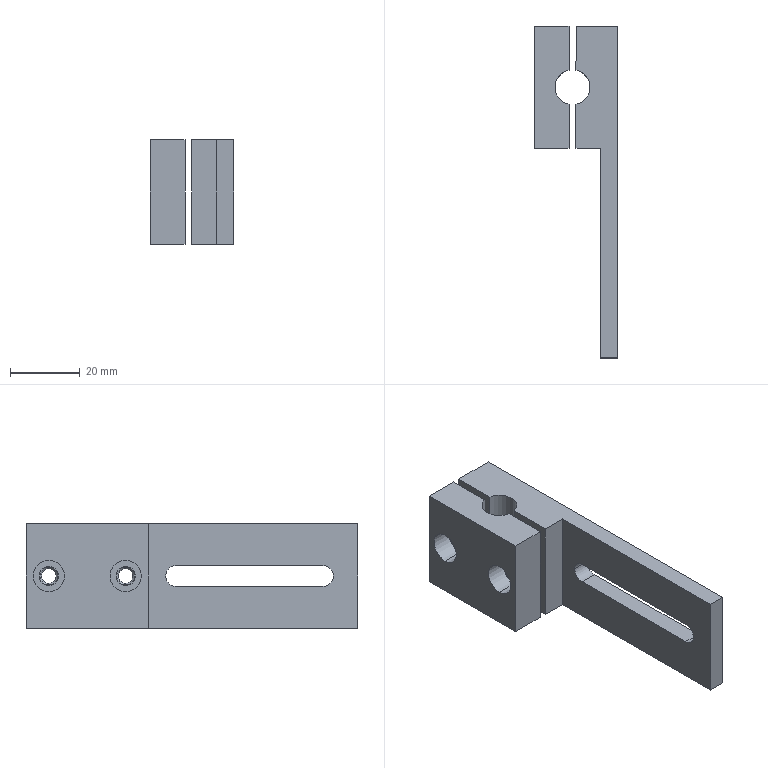Component | SolidWorks | PhotoelectricBracket-1 | 2 solids | 41 faces | volume 27650 mm3 | plane 20 | cylinder 17 | cone 4 | commonest cylinder face diameters 9 x4 5.5 x4 4.2 x4 6 x3 10 x2